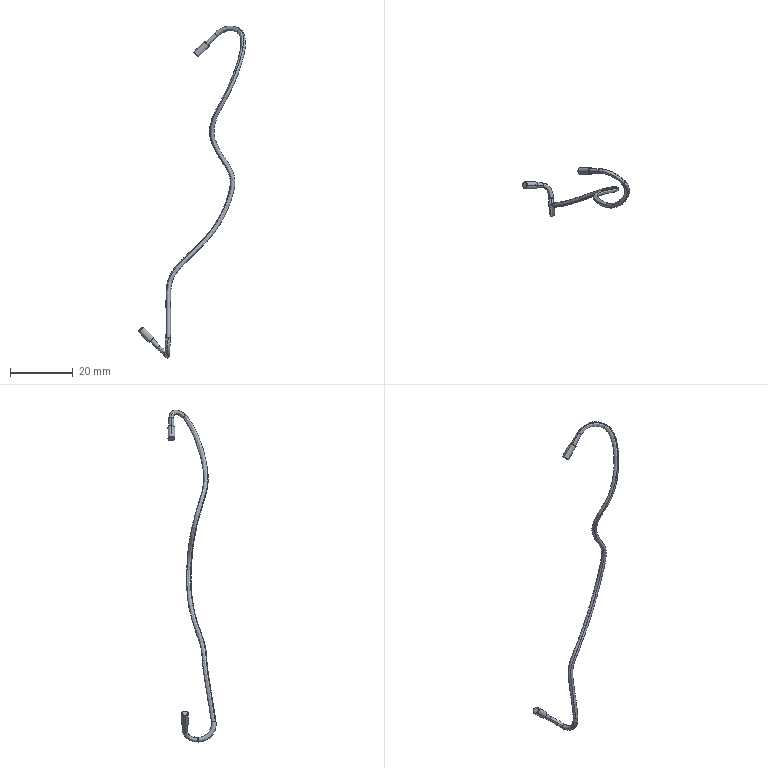Component | SolidWorks | Crijevo_paX3-1 | 3 solids | 56 faces | box 34.22 x 15.45 x 106.17 mm | volume 98 mm3 | cylinder 20 | torus 16 | plane 8 | spline 8 | cone 4 | commonest cylinder face diameters 1.5 x10 1.3 x6 2.2 x4